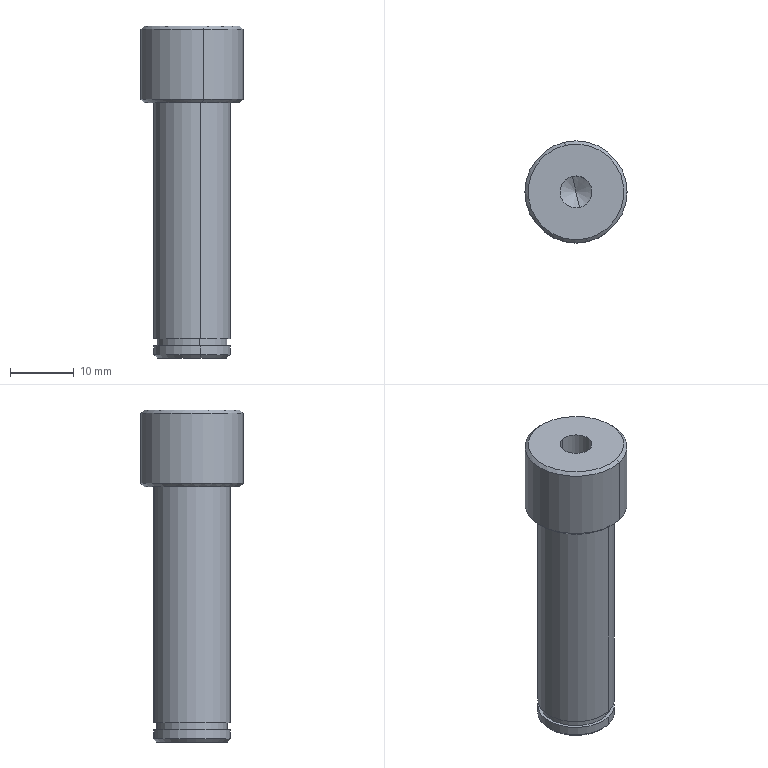Component | SolidWorks | JYTBJ-HeaderBrakeAxis-1 | 1 solid | 23 faces | box 16 x 16 x 52 mm | volume 6556 mm3 | cylinder 10 | cone 8 | plane 5 | commonest cylinder face diameters 12 x4 11 x2 5 x2 16 x2 | material AISI 1045 Steel, Cold Drawn
build123d program:
from build123d import *

# Parameters (mm, degrees)
SKETCH1_R             = 6
BOSS_EXTRUDE1_DEPTH   = 20
SKETCH2_R             = 8
BOSS_EXTRUDE2_DEPTH   = 12
M6_TAPPED_HOLE1_D     = 5
M6_TAPPED_HOLE1_DEPTH = 17
M6_TAPPED_HOLE1_TIP   = 1.502
SKETCH6_W             = 8.155
SKETCH6_H             = 1.1
CHAMFER1_SIZE         = 0.5


with BuildPart() as part:
    # Sketch1 → Boss-Extrude1 (new, symmetric)
    with BuildSketch(Plane.XY):
        Circle(SKETCH1_R)
    extrude(amount=BOSS_EXTRUDE1_DEPTH, both=True)

    # Sketch2 → Boss-Extrude2 (add)
    with BuildSketch(Plane.XY.offset(20)):
        Circle(SKETCH2_R)
    extrude(amount=BOSS_EXTRUDE2_DEPTH)

    # M6 Tapped Hole1
    with Locations(Plane(origin=(-7.558, 9.246, 32), x_dir=(1, 0, 0), z_dir=(0, 0, 1))):
        with Locations((7.558, -9.246)):
            Hole(M6_TAPPED_HOLE1_D / 2, depth=M6_TAPPED_HOLE1_DEPTH)
            with Locations((0, 0, -(M6_TAPPED_HOLE1_DEPTH + M6_TAPPED_HOLE1_TIP / 2))):  # 118° drill point
                Cone(0, M6_TAPPED_HOLE1_D / 2, M6_TAPPED_HOLE1_TIP, mode=Mode.SUBTRACT)

    # Sketch6 → Cut-Revolve1 (revolve, cut)
    with BuildSketch(Plane(origin=(0, 0, 0), x_dir=(1, 0, 0), z_dir=(0, 1, 0))):
        with Locations((9.578, 17.55)):
            Rectangle(SKETCH6_W, SKETCH6_H)
    revolve(axis=Axis((0, 0, 20), (0, 0, -1)), mode=Mode.SUBTRACT)

    # Chamfer1
    chamfer1_edges = [part.edges().sort_by_distance(p)[0] for p in [
        (-6, 0, -20),
        (-8, 0, 20),
        (-8, 0, 32),
    ]]
    chamfer(chamfer1_edges, length=CHAMFER1_SIZE)


solid = part.part

# Placed as in the assembly
solid = solid.moved(Location((-71.627, 226.781, -21), (0, 0, 0)))
STEP:
#1=COLOUR_RGB('',0.7922,0.8196,0.9333);
#2=FILL_AREA_STYLE_COLOUR('',#1);
#3=FILL_AREA_STYLE('',(#2));
#4=SURFACE_STYLE_FILL_AREA(#3);
#5=SURFACE_SIDE_STYLE('',(#4));
#6=SURFACE_STYLE_USAGE(.BOTH.,#5);
#7=PRESENTATION_STYLE_ASSIGNMENT((#6));
#8=CARTESIAN_POINT('',(-2.868,9.139,-1.614));
#9=VERTEX_POINT('',#8);
#10=CARTESIAN_POINT('',(-2.772,8.717,-1.614));
#11=VERTEX_POINT('',#10);
#12=CARTESIAN_POINT('',(-2.82,8.928,-1.614));
#13=DIRECTION('',(-0.,0.,-1.));
#14=DIRECTION('',(0.2228,-0.9749,0.));
#15=AXIS2_PLACEMENT_3D('',#12,#13,#14);
#16=CIRCLE('',#15,0.2165);
#17=EDGE_CURVE('',#9,#11,#16,.T.);
#18=ORIENTED_EDGE('',*,*,#17,.F.);
#19=CARTESIAN_POINT('',(-2.873,9.159,-1.594));
#20=VERTEX_POINT('',#19);
#21=CARTESIAN_POINT('',(-2.873,9.159,-1.594));
#22=DIRECTION('',(-0.1576,0.6893,0.7071));
#23=VECTOR('',#22,39.37);
#24=LINE('',#21,#23);
#25=EDGE_CURVE('',#9,#20,#24,.T.);
#26=ORIENTED_EDGE('',*,*,#25,.T.);
#27=CARTESIAN_POINT('',(-2.767,8.698,-1.594));
#28=VERTEX_POINT('',#27);
#29=CARTESIAN_POINT('',(-2.82,8.928,-1.594));
#30=DIRECTION('',(0.,-0.,1.));
#31=DIRECTION('',(0.2228,-0.9749,0.));
#32=AXIS2_PLACEMENT_3D('',#29,#30,#31);
#33=CIRCLE('',#32,0.2362);
#34=EDGE_CURVE('',#28,#20,#33,.T.);
#35=ORIENTED_EDGE('',*,*,#34,.F.);
#36=CARTESIAN_POINT('',(-2.767,8.698,-1.594));
#37=DIRECTION('',(0.1576,-0.6893,0.7071));
#38=VECTOR('',#37,39.37);
#39=LINE('',#36,#38);
#40=EDGE_CURVE('',#11,#28,#39,.T.);
#41=ORIENTED_EDGE('',*,*,#40,.F.);
#42=EDGE_LOOP('',(#18,#26,#35,#41));
#43=FACE_OUTER_BOUND('',#42,.T.);
#44=CARTESIAN_POINT('',(-2.82,8.928,-1.594));
#45=DIRECTION('',(0.,-0.,1.));
#46=DIRECTION('',(0.2228,-0.9749,0.));
#47=AXIS2_PLACEMENT_3D('',#44,#45,#46);
#48=CONICAL_SURFACE('',#47,0.2362,0.7854);
#49=ADVANCED_FACE('',(#43),#48,.T.);
#50=CARTESIAN_POINT('',(-2.886,9.216,-0.03937));
#51=VERTEX_POINT('',#50);
#52=CARTESIAN_POINT('',(-2.754,8.641,-0.03937));
#53=VERTEX_POINT('',#52);
#54=CARTESIAN_POINT('',(-2.82,8.928,-0.03937));
#55=DIRECTION('',(-0.,0.,-1.));
#56=DIRECTION('',(0.2228,-0.9749,0.));
#57=AXIS2_PLACEMENT_3D('',#54,#55,#56);
#58=CIRCLE('',#57,0.2953);
#59=EDGE_CURVE('',#51,#53,#58,.T.);
#60=ORIENTED_EDGE('',*,*,#59,.F.);
#61=CARTESIAN_POINT('',(-2.89,9.235,-0.01969));
#62=VERTEX_POINT('',#61);
#63=CARTESIAN_POINT('',(-2.89,9.235,-0.01969));
#64=DIRECTION('',(-0.1576,0.6893,0.7071));
#65=VECTOR('',#64,39.37);
#66=LINE('',#63,#65);
#67=EDGE_CURVE('',#51,#62,#66,.T.);
#68=ORIENTED_EDGE('',*,*,#67,.T.);
#69=CARTESIAN_POINT('',(-2.75,8.621,-0.01969));
#70=VERTEX_POINT('',#69);
#71=CARTESIAN_POINT('',(-2.82,8.928,-0.01969));
#72=DIRECTION('',(0.,-0.,1.));
#73=DIRECTION('',(0.2228,-0.9749,0.));
#74=AXIS2_PLACEMENT_3D('',#71,#72,#73);
#75=CIRCLE('',#74,0.315);
#76=EDGE_CURVE('',#70,#62,#75,.T.);
#77=ORIENTED_EDGE('',*,*,#76,.F.);
#78=CARTESIAN_POINT('',(-2.75,8.621,-0.01969));
#79=DIRECTION('',(0.1576,-0.6893,0.7071));
#80=VECTOR('',#79,39.37);
#81=LINE('',#78,#80);
#82=EDGE_CURVE('',#53,#70,#81,.T.);
#83=ORIENTED_EDGE('',*,*,#82,.F.);
#84=EDGE_LOOP('',(#60,#68,#77,#83));
#85=FACE_OUTER_BOUND('',#84,.T.);
#86=CARTESIAN_POINT('',(-2.82,8.928,-0.01969));
#87=DIRECTION('',(0.,-0.,1.));
#88=DIRECTION('',(0.2228,-0.9749,0.));
#89=AXIS2_PLACEMENT_3D('',#86,#87,#88);
#90=CONICAL_SURFACE('',#89,0.315,0.7854);
#91=ADVANCED_FACE('',(#85),#90,.T.);
#92=CARTESIAN_POINT('',(-2.754,8.641,0.4331));
#93=VERTEX_POINT('',#92);
#94=CARTESIAN_POINT('',(-2.886,9.216,0.4331));
#95=VERTEX_POINT('',#94);
#96=CARTESIAN_POINT('',(-2.82,8.928,0.4331));
#97=DIRECTION('',(0.,-0.,1.));
#98=DIRECTION('',(0.2228,-0.9749,0.));
#99=AXIS2_PLACEMENT_3D('',#96,#97,#98);
#100=CIRCLE('',#99,0.2953);
#101=EDGE_CURVE('',#93,#95,#100,.T.);
#102=ORIENTED_EDGE('',*,*,#101,.F.);
#103=CARTESIAN_POINT('',(-2.75,8.621,0.4134));
#104=VERTEX_POINT('',#103);
#105=CARTESIAN_POINT('',(-2.754,8.641,0.4331));
#106=DIRECTION('',(0.1576,-0.6893,-0.7071));
#107=VECTOR('',#106,39.37);
#108=LINE('',#105,#107);
#109=EDGE_CURVE('',#93,#104,#108,.T.);
#110=ORIENTED_EDGE('',*,*,#109,.T.);
#111=CARTESIAN_POINT('',(-2.89,9.235,0.4134));
#112=VERTEX_POINT('',#111);
#113=CARTESIAN_POINT('',(-2.82,8.928,0.4134));
#114=DIRECTION('',(-0.,0.,-1.));
#115=DIRECTION('',(0.2228,-0.9749,0.));
#116=AXIS2_PLACEMENT_3D('',#113,#114,#115);
#117=CIRCLE('',#116,0.315);
#118=EDGE_CURVE('',#112,#104,#117,.T.);
#119=ORIENTED_EDGE('',*,*,#118,.F.);
#120=CARTESIAN_POINT('',(-2.886,9.216,0.4331));
#121=DIRECTION('',(-0.1576,0.6893,-0.7071));
#122=VECTOR('',#121,39.37);
#123=LINE('',#120,#122);
#124=EDGE_CURVE('',#95,#112,#123,.T.);
#125=ORIENTED_EDGE('',*,*,#124,.F.);
#126=EDGE_LOOP('',(#102,#110,#119,#125));
#127=FACE_OUTER_BOUND('',#126,.T.);
#128=CARTESIAN_POINT('',(-2.82,8.928,0.4331));
#129=DIRECTION('',(-0.,0.,-1.));
#130=DIRECTION('',(-0.2228,0.9749,0.));
#131=AXIS2_PLACEMENT_3D('',#128,#129,#130);
#132=CONICAL_SURFACE('',#131,0.2953,0.7854);
#133=ADVANCED_FACE('',(#127),#132,.T.);
#134=CARTESIAN_POINT('',(-2.873,9.159,-1.539));
#135=VERTEX_POINT('',#134);
#136=CARTESIAN_POINT('',(-2.767,8.698,-1.539));
#137=VERTEX_POINT('',#136);
#138=CARTESIAN_POINT('',(-2.82,8.928,-1.539));
#139=DIRECTION('',(-0.,0.,-1.));
#140=DIRECTION('',(-0.2228,0.9749,0.));
#141=AXIS2_PLACEMENT_3D('',#138,#139,#140);
#142=CIRCLE('',#141,0.2362);
#143=EDGE_CURVE('',#135,#137,#142,.T.);
#144=ORIENTED_EDGE('',*,*,#143,.T.);
#145=CARTESIAN_POINT('',(-2.767,8.698,-0.03937));
#146=DIRECTION('',(-0.,0.,-1.));
#147=VECTOR('',#146,39.37);
#148=LINE('',#145,#147);
#149=EDGE_CURVE('',#137,#28,#148,.T.);
#150=ORIENTED_EDGE('',*,*,#149,.T.);
#151=ORIENTED_EDGE('',*,*,#34,.T.);
#152=CARTESIAN_POINT('',(-2.873,9.159,-0.03937));
#153=DIRECTION('',(-0.,0.,-1.));
#154=VECTOR('',#153,39.37);
#155=LINE('',#152,#154);
#156=EDGE_CURVE('',#135,#20,#155,.T.);
#157=ORIENTED_EDGE('',*,*,#156,.F.);
#158=EDGE_LOOP('',(#144,#150,#151,#157));
#159=FACE_OUTER_BOUND('',#158,.T.);
#160=CARTESIAN_POINT('',(-2.82,8.928,-0.03937));
#161=DIRECTION('',(-0.,0.,-1.));
#162=DIRECTION('',(-0.2228,0.9749,0.));
#163=AXIS2_PLACEMENT_3D('',#160,#161,#162);
#164=CYLINDRICAL_SURFACE('',#163,0.2362);
#165=ADVANCED_FACE('',(#159),#164,.T.);
#166=CARTESIAN_POINT('',(-2.772,8.717,-1.539));
#167=VERTEX_POINT('',#166);
#168=CARTESIAN_POINT('',(-2.868,9.139,-1.539));
#169=VERTEX_POINT('',#168);
#170=CARTESIAN_POINT('',(-2.82,8.928,-1.539));
#171=DIRECTION('',(0.,-0.,1.));
#172=DIRECTION('',(0.2228,-0.9749,0.));
#173=AXIS2_PLACEMENT_3D('',#170,#171,#172);
#174=CIRCLE('',#173,0.2165);
#175=EDGE_CURVE('',#167,#169,#174,.T.);
#176=ORIENTED_EDGE('',*,*,#175,.T.);
#177=CARTESIAN_POINT('',(-2.868,9.139,-1.496));
#178=VERTEX_POINT('',#177);
#179=CARTESIAN_POINT('',(-2.868,9.139,-0.03937));
#180=DIRECTION('',(0.,-0.,1.));
#181=VECTOR('',#180,39.37);
#182=LINE('',#179,#181);
#183=EDGE_CURVE('',#169,#178,#182,.T.);
#184=ORIENTED_EDGE('',*,*,#183,.T.);
#185=CARTESIAN_POINT('',(-2.772,8.717,-1.496));
#186=VERTEX_POINT('',#185);
#187=CARTESIAN_POINT('',(-2.82,8.928,-1.496));
#188=DIRECTION('',(0.,-0.,1.));
#189=DIRECTION('',(0.2228,-0.9749,0.));
#190=AXIS2_PLACEMENT_3D('',#187,#188,#189);
#191=CIRCLE('',#190,0.2165);
#192=EDGE_CURVE('',#186,#178,#191,.T.);
#193=ORIENTED_EDGE('',*,*,#192,.F.);
#194=CARTESIAN_POINT('',(-2.772,8.717,-0.03937));
#195=DIRECTION('',(0.,-0.,1.));
#196=VECTOR('',#195,39.37);
#197=LINE('',#194,#196);
#198=EDGE_CURVE('',#167,#186,#197,.T.);
#199=ORIENTED_EDGE('',*,*,#198,.F.);
#200=EDGE_LOOP('',(#176,#184,#193,#199));
#201=FACE_OUTER_BOUND('',#200,.T.);
#202=CARTESIAN_POINT('',(-2.82,8.928,-0.03937));
#203=DIRECTION('',(0.,-0.,1.));
#204=DIRECTION('',(0.2228,-0.9749,0.));
#205=AXIS2_PLACEMENT_3D('',#202,#203,#204);
#206=CYLINDRICAL_SURFACE('',#205,0.2165);
#207=ADVANCED_FACE('',(#201),#206,.T.);
#208=CARTESIAN_POINT('',(-2.842,9.024,-0.2362));
#209=VERTEX_POINT('',#208);
#210=CARTESIAN_POINT('',(-2.798,8.832,-0.2362));
#211=VERTEX_POINT('',#210);
#212=CARTESIAN_POINT('',(-2.82,8.928,-0.2362));
#213=DIRECTION('',(0.,-0.,1.));
#214=DIRECTION('',(0.2228,-0.9749,0.));
#215=AXIS2_PLACEMENT_3D('',#212,#213,#214);
#216=CIRCLE('',#215,0.09843);
#217=EDGE_CURVE('',#209,#211,#216,.T.);
#218=ORIENTED_EDGE('',*,*,#217,.F.);
#219=CARTESIAN_POINT('',(-2.842,9.024,0.4331));
#220=VERTEX_POINT('',#219);
#221=CARTESIAN_POINT('',(-2.842,9.024,0.4331));
#222=DIRECTION('',(0.,-0.,1.));
#223=VECTOR('',#222,39.37);
#224=LINE('',#221,#223);
#225=EDGE_CURVE('',#209,#220,#224,.T.);
#226=ORIENTED_EDGE('',*,*,#225,.T.);
#227=CARTESIAN_POINT('',(-2.798,8.832,0.4331));
#228=VERTEX_POINT('',#227);
#229=CARTESIAN_POINT('',(-2.82,8.928,0.4331));
#230=DIRECTION('',(0.,-0.,1.));
#231=DIRECTION('',(0.2228,-0.9749,0.));
#232=AXIS2_PLACEMENT_3D('',#229,#230,#231);
#233=CIRCLE('',#232,0.09843);
#234=EDGE_CURVE('',#220,#228,#233,.T.);
#235=ORIENTED_EDGE('',*,*,#234,.T.);
#236=CARTESIAN_POINT('',(-2.798,8.832,0.4331));
#237=DIRECTION('',(0.,-0.,1.));
#238=VECTOR('',#237,39.37);
#239=LINE('',#236,#238);
#240=EDGE_CURVE('',#211,#228,#239,.T.);
#241=ORIENTED_EDGE('',*,*,#240,.F.);
#242=EDGE_LOOP('',(#218,#226,#235,#241));
#243=FACE_OUTER_BOUND('',#242,.T.);
#244=CARTESIAN_POINT('',(-2.82,8.928,0.4331));
#245=DIRECTION('',(0.,-0.,1.));
#246=DIRECTION('',(0.2228,-0.9749,0.));
#247=AXIS2_PLACEMENT_3D('',#244,#245,#246);
#248=CYLINDRICAL_SURFACE('',#247,0.09843);
#249=ADVANCED_FACE('',(#243),#248,.F.);
#250=CARTESIAN_POINT('',(-2.82,8.928,-0.2954));
#251=VERTEX_POINT('',#250);
#252=CARTESIAN_POINT('',(-2.798,8.832,-0.2362));
#253=DIRECTION('',(0.191,-0.8356,0.515));
#254=VECTOR('',#253,39.37);
#255=LINE('',#252,#254);
#256=EDGE_CURVE('',#251,#211,#255,.T.);
#257=ORIENTED_EDGE('',*,*,#256,.F.);
#258=CARTESIAN_POINT('',(-2.842,9.024,-0.2362));
#259=DIRECTION('',(-0.191,0.8356,0.515));
#260=VECTOR('',#259,39.37);
#261=LINE('',#258,#260);
#262=EDGE_CURVE('',#251,#209,#261,.T.);
#263=ORIENTED_EDGE('',*,*,#262,.T.);
#264=ORIENTED_EDGE('',*,*,#217,.T.);
#265=EDGE_LOOP('',(#257,#263,#264));
#266=FACE_OUTER_BOUND('',#265,.T.);
#267=CARTESIAN_POINT('',(-2.82,8.928,-0.2362));
#268=DIRECTION('',(0.,-0.,1.));
#269=DIRECTION('',(0.2228,-0.9749,0.));
#270=AXIS2_PLACEMENT_3D('',#267,#268,#269);
#271=CONICAL_SURFACE('',#270,0.09843,1.03);
#272=ADVANCED_FACE('',(#266),#271,.F.);
#273=ORIENTED_EDGE('',*,*,#118,.T.);
#274=CARTESIAN_POINT('',(-2.75,8.621,0.4331));
#275=DIRECTION('',(-0.,0.,-1.));
#276=VECTOR('',#275,39.37);
#277=LINE('',#274,#276);
#278=EDGE_CURVE('',#104,#70,#277,.T.);
#279=ORIENTED_EDGE('',*,*,#278,.T.);
#280=ORIENTED_EDGE('',*,*,#76,.T.);
#281=CARTESIAN_POINT('',(-2.89,9.235,0.4331));
#282=DIRECTION('',(-0.,0.,-1.));
#283=VECTOR('',#282,39.37);
#284=LINE('',#281,#283);
#285=EDGE_CURVE('',#112,#62,#284,.T.);
#286=ORIENTED_EDGE('',*,*,#285,.F.);
#287=EDGE_LOOP('',(#273,#279,#280,#286));
#288=FACE_OUTER_BOUND('',#287,.T.);
#289=CARTESIAN_POINT('',(-2.82,8.928,0.4331));
#290=DIRECTION('',(-0.,0.,-1.));
#291=DIRECTION('',(-0.2228,0.9749,0.));
#292=AXIS2_PLACEMENT_3D('',#289,#290,#291);
#293=CYLINDRICAL_SURFACE('',#292,0.315);
#294=ADVANCED_FACE('',(#288),#293,.T.);
#295=CARTESIAN_POINT('',(-2.767,8.698,-0.03937));
#296=VERTEX_POINT('',#295);
#297=CARTESIAN_POINT('',(-2.873,9.159,-0.03937));
#298=VERTEX_POINT('',#297);
#299=CARTESIAN_POINT('',(-2.82,8.928,-0.03937));
#300=DIRECTION('',(0.,-0.,1.));
#301=DIRECTION('',(0.2228,-0.9749,0.));
#302=AXIS2_PLACEMENT_3D('',#299,#300,#301);
#303=CIRCLE('',#302,0.2362);
#304=EDGE_CURVE('',#296,#298,#303,.T.);
#305=ORIENTED_EDGE('',*,*,#304,.F.);
#306=CARTESIAN_POINT('',(-2.767,8.698,-1.496));
#307=VERTEX_POINT('',#306);
#308=CARTESIAN_POINT('',(-2.767,8.698,-0.03937));
#309=DIRECTION('',(-0.,0.,-1.));
#310=VECTOR('',#309,39.37);
#311=LINE('',#308,#310);
#312=EDGE_CURVE('',#296,#307,#311,.T.);
#313=ORIENTED_EDGE('',*,*,#312,.T.);
#314=CARTESIAN_POINT('',(-2.873,9.159,-1.496));
#315=VERTEX_POINT('',#314);
#316=CARTESIAN_POINT('',(-2.82,8.928,-1.496));
#317=DIRECTION('',(0.,-0.,1.));
#318=DIRECTION('',(0.2228,-0.9749,0.));
#319=AXIS2_PLACEMENT_3D('',#316,#317,#318);
#320=CIRCLE('',#319,0.2362);
#321=EDGE_CURVE('',#307,#315,#320,.T.);
#322=ORIENTED_EDGE('',*,*,#321,.T.);
#323=CARTESIAN_POINT('',(-2.873,9.159,-0.03937));
#324=DIRECTION('',(-0.,0.,-1.));
#325=VECTOR('',#324,39.37);
#326=LINE('',#323,#325);
#327=EDGE_CURVE('',#298,#315,#326,.T.);
#328=ORIENTED_EDGE('',*,*,#327,.F.);
#329=EDGE_LOOP('',(#305,#313,#322,#328));
#330=FACE_OUTER_BOUND('',#329,.T.);
#331=CARTESIAN_POINT('',(-2.82,8.928,-0.03937));
#332=DIRECTION('',(-0.,0.,-1.));
#333=DIRECTION('',(-0.2228,0.9749,0.));
#334=AXIS2_PLACEMENT_3D('',#331,#332,#333);
#335=CYLINDRICAL_SURFACE('',#334,0.2362);
#336=ADVANCED_FACE('',(#330),#335,.T.);
#337=ORIENTED_EDGE('',*,*,#312,.F.);
#338=CARTESIAN_POINT('',(-2.82,8.928,-0.03937));
#339=DIRECTION('',(0.,-0.,1.));
#340=DIRECTION('',(0.2228,-0.9749,0.));
#341=AXIS2_PLACEMENT_3D('',#338,#339,#340);
#342=CIRCLE('',#341,0.2362);
#343=EDGE_CURVE('',#298,#296,#342,.T.);
#344=ORIENTED_EDGE('',*,*,#343,.F.);
#345=ORIENTED_EDGE('',*,*,#327,.T.);
#346=CARTESIAN_POINT('',(-2.82,8.928,-1.496));
#347=DIRECTION('',(0.,-0.,1.));
#348=DIRECTION('',(0.2228,-0.9749,0.));
#349=AXIS2_PLACEMENT_3D('',#346,#347,#348);
#350=CIRCLE('',#349,0.2362);
#351=EDGE_CURVE('',#315,#307,#350,.T.);
#352=ORIENTED_EDGE('',*,*,#351,.T.);
#353=EDGE_LOOP('',(#337,#344,#345,#352));
#354=FACE_OUTER_BOUND('',#353,.T.);
#355=CARTESIAN_POINT('',(-2.82,8.928,-0.03937));
#356=DIRECTION('',(-0.,0.,-1.));
#357=DIRECTION('',(-0.2228,0.9749,0.));
#358=AXIS2_PLACEMENT_3D('',#355,#356,#357);
#359=CYLINDRICAL_SURFACE('',#358,0.2362);
#360=ADVANCED_FACE('',(#354),#359,.T.);
#361=CARTESIAN_POINT('',(-2.82,8.928,-0.03937));
#362=DIRECTION('',(-0.,0.,-1.));
#363=DIRECTION('',(0.2228,-0.9749,0.));
#364=AXIS2_PLACEMENT_3D('',#361,#362,#363);
#365=CIRCLE('',#364,0.2953);
#366=EDGE_CURVE('',#53,#51,#365,.T.);
#367=ORIENTED_EDGE('',*,*,#366,.T.);
#368=ORIENTED_EDGE('',*,*,#59,.T.);
#369=EDGE_LOOP('',(#367,#368));
#370=FACE_OUTER_BOUND('',#369,.T.);
#371=ORIENTED_EDGE('',*,*,#343,.T.);
#372=ORIENTED_EDGE('',*,*,#304,.T.);
#373=EDGE_LOOP('',(#371,#372));
#374=FACE_BOUND('',#373,.T.);
#375=CARTESIAN_POINT('',(-2.82,8.928,-0.03937));
#376=DIRECTION('',(0.,-0.,1.));
#377=DIRECTION('',(0.2228,-0.9749,-0.));
#378=AXIS2_PLACEMENT_3D('',#375,#376,#377);
#379=PLANE('',#378);
#380=ADVANCED_FACE('',(#370,#374),#379,.F.);
#381=ORIENTED_EDGE('',*,*,#278,.F.);
#382=CARTESIAN_POINT('',(-2.82,8.928,0.4134));
#383=DIRECTION('',(-0.,0.,-1.));
#384=DIRECTION('',(0.2228,-0.9749,0.));
#385=AXIS2_PLACEMENT_3D('',#382,#383,#384);
#386=CIRCLE('',#385,0.315);
#387=EDGE_CURVE('',#104,#112,#386,.T.);
#388=ORIENTED_EDGE('',*,*,#387,.T.);
#389=ORIENTED_EDGE('',*,*,#285,.T.);
#390=CARTESIAN_POINT('',(-2.82,8.928,-0.01969));
#391=DIRECTION('',(0.,-0.,1.));
#392=DIRECTION('',(0.2228,-0.9749,0.));
#393=AXIS2_PLACEMENT_3D('',#390,#391,#392);
#394=CIRCLE('',#393,0.315);
#395=EDGE_CURVE('',#62,#70,#394,.T.);
#396=ORIENTED_EDGE('',*,*,#395,.T.);
#397=EDGE_LOOP('',(#381,#388,#389,#396));
#398=FACE_OUTER_BOUND('',#397,.T.);
#399=CARTESIAN_POINT('',(-2.82,8.928,0.4331));
#400=DIRECTION('',(-0.,0.,-1.));
#401=DIRECTION('',(-0.2228,0.9749,0.));
#402=AXIS2_PLACEMENT_3D('',#399,#400,#401);
#403=CYLINDRICAL_SURFACE('',#402,0.315);
#404=ADVANCED_FACE('',(#398),#403,.T.);
#405=CARTESIAN_POINT('',(-2.82,8.928,0.4331));
#406=DIRECTION('',(0.,-0.,1.));
#407=DIRECTION('',(0.2228,-0.9749,0.));
#408=AXIS2_PLACEMENT_3D('',#405,#406,#407);
#409=CIRCLE('',#408,0.2953);
#410=EDGE_CURVE('',#95,#93,#409,.T.);
#411=ORIENTED_EDGE('',*,*,#410,.T.);
#412=ORIENTED_EDGE('',*,*,#101,.T.);
#413=EDGE_LOOP('',(#411,#412));
#414=FACE_OUTER_BOUND('',#413,.T.);
#415=CARTESIAN_POINT('',(-2.82,8.928,0.4331));
#416=DIRECTION('',(0.,-0.,1.));
#417=DIRECTION('',(0.2228,-0.9749,0.));
#418=AXIS2_PLACEMENT_3D('',#415,#416,#417);
#419=CIRCLE('',#418,0.09843);
#420=EDGE_CURVE('',#228,#220,#419,.T.);
#421=ORIENTED_EDGE('',*,*,#420,.F.);
#422=ORIENTED_EDGE('',*,*,#234,.F.);
#423=EDGE_LOOP('',(#421,#422));
#424=FACE_BOUND('',#423,.T.);
#425=CARTESIAN_POINT('',(-2.82,8.928,0.4331));
#426=DIRECTION('',(0.,-0.,1.));
#427=DIRECTION('',(0.2228,-0.9749,-0.));
#428=AXIS2_PLACEMENT_3D('',#425,#426,#427);
#429=PLANE('',#428);
#430=ADVANCED_FACE('',(#414,#424),#429,.T.);
#431=ORIENTED_EDGE('',*,*,#262,.F.);
#432=ORIENTED_EDGE('',*,*,#256,.T.);
#433=CARTESIAN_POINT('',(-2.82,8.928,-0.2362));
#434=DIRECTION('',(0.,-0.,1.));
#435=DIRECTION('',(0.2228,-0.9749,0.));
#436=AXIS2_PLACEMENT_3D('',#433,#434,#435);
#437=CIRCLE('',#436,0.09843);
#438=EDGE_CURVE('',#211,#209,#437,.T.);
#439=ORIENTED_EDGE('',*,*,#438,.T.);
#440=EDGE_LOOP('',(#431,#432,#439));
#441=FACE_OUTER_BOUND('',#440,.T.);
#442=CARTESIAN_POINT('',(-2.82,8.928,-0.2362));
#443=DIRECTION('',(0.,-0.,1.));
#444=DIRECTION('',(0.2228,-0.9749,0.));
#445=AXIS2_PLACEMENT_3D('',#442,#443,#444);
#446=CONICAL_SURFACE('',#445,0.09843,1.03);
#447=ADVANCED_FACE('',(#441),#446,.F.);
#448=ORIENTED_EDGE('',*,*,#225,.F.);
#449=ORIENTED_EDGE('',*,*,#438,.F.);
#450=ORIENTED_EDGE('',*,*,#240,.T.);
#451=ORIENTED_EDGE('',*,*,#420,.T.);
#452=EDGE_LOOP('',(#448,#449,#450,#451));
#453=FACE_OUTER_BOUND('',#452,.T.);
#454=CARTESIAN_POINT('',(-2.82,8.928,0.4331));
#455=DIRECTION('',(0.,-0.,1.));
#456=DIRECTION('',(0.2228,-0.9749,0.));
#457=AXIS2_PLACEMENT_3D('',#454,#455,#456);
#458=CYLINDRICAL_SURFACE('',#457,0.09843);
#459=ADVANCED_FACE('',(#453),#458,.F.);
#460=ORIENTED_EDGE('',*,*,#192,.T.);
#461=CARTESIAN_POINT('',(-2.82,8.928,-1.496));
#462=DIRECTION('',(0.,-0.,1.));
#463=DIRECTION('',(0.2228,-0.9749,0.));
#464=AXIS2_PLACEMENT_3D('',#461,#462,#463);
#465=CIRCLE('',#464,0.2165);
#466=EDGE_CURVE('',#178,#186,#465,.T.);
#467=ORIENTED_EDGE('',*,*,#466,.T.);
#468=EDGE_LOOP('',(#460,#467));
#469=FACE_BOUND('',#468,.T.);
#470=ORIENTED_EDGE('',*,*,#351,.F.);
#471=ORIENTED_EDGE('',*,*,#321,.F.);
#472=EDGE_LOOP('',(#470,#471));
#473=FACE_OUTER_BOUND('',#472,.T.);
#474=CARTESIAN_POINT('',(-2.772,8.717,-1.496));
#475=DIRECTION('',(0.,-0.,1.));
#476=DIRECTION('',(0.2228,-0.9749,-0.));
#477=AXIS2_PLACEMENT_3D('',#474,#475,#476);
#478=PLANE('',#477);
#479=ADVANCED_FACE('',(#469,#473),#478,.F.);
#480=ORIENTED_EDGE('',*,*,#175,.F.);
#481=CARTESIAN_POINT('',(-2.82,8.928,-1.539));
#482=DIRECTION('',(0.,-0.,1.));
#483=DIRECTION('',(0.2228,-0.9749,0.));
#484=AXIS2_PLACEMENT_3D('',#481,#482,#483);
#485=CIRCLE('',#484,0.2165);
#486=EDGE_CURVE('',#169,#167,#485,.T.);
#487=ORIENTED_EDGE('',*,*,#486,.F.);
#488=EDGE_LOOP('',(#480,#487));
#489=FACE_BOUND('',#488,.T.);
#490=ORIENTED_EDGE('',*,*,#143,.F.);
#491=CARTESIAN_POINT('',(-2.82,8.928,-1.539));
#492=DIRECTION('',(-0.,0.,-1.));
#493=DIRECTION('',(-0.2228,0.9749,0.));
#494=AXIS2_PLACEMENT_3D('',#491,#492,#493);
#495=CIRCLE('',#494,0.2362);
#496=EDGE_CURVE('',#137,#135,#495,.T.);
#497=ORIENTED_EDGE('',*,*,#496,.F.);
#498=EDGE_LOOP('',(#490,#497));
#499=FACE_OUTER_BOUND('',#498,.T.);
#500=CARTESIAN_POINT('',(-2.772,8.717,-1.539));
#501=DIRECTION('',(-0.,0.,-1.));
#502=DIRECTION('',(-0.2228,0.9749,0.));
#503=AXIS2_PLACEMENT_3D('',#500,#501,#502);
#504=PLANE('',#503);
#505=ADVANCED_FACE('',(#489,#499),#504,.F.);
#506=ORIENTED_EDGE('',*,*,#183,.F.);
#507=ORIENTED_EDGE('',*,*,#486,.T.);
#508=ORIENTED_EDGE('',*,*,#198,.T.);
#509=ORIENTED_EDGE('',*,*,#466,.F.);
#510=EDGE_LOOP('',(#506,#507,#508,#509));
#511=FACE_OUTER_BOUND('',#510,.T.);
#512=CARTESIAN_POINT('',(-2.82,8.928,-0.03937));
#513=DIRECTION('',(0.,-0.,1.));
#514=DIRECTION('',(0.2228,-0.9749,0.));
#515=AXIS2_PLACEMENT_3D('',#512,#513,#514);
#516=CYLINDRICAL_SURFACE('',#515,0.2165);
#517=ADVANCED_FACE('',(#511),#516,.T.);
#518=CARTESIAN_POINT('',(-2.82,8.928,-1.614));
#519=DIRECTION('',(-0.,0.,-1.));
#520=DIRECTION('',(0.2228,-0.9749,0.));
#521=AXIS2_PLACEMENT_3D('',#518,#519,#520);
#522=CIRCLE('',#521,0.2165);
#523=EDGE_CURVE('',#11,#9,#522,.T.);
#524=ORIENTED_EDGE('',*,*,#523,.T.);
#525=ORIENTED_EDGE('',*,*,#17,.T.);
#526=EDGE_LOOP('',(#524,#525));
#527=FACE_OUTER_BOUND('',#526,.T.);
#528=CARTESIAN_POINT('',(-2.82,8.928,-1.614));
#529=DIRECTION('',(0.,-0.,1.));
#530=DIRECTION('',(0.2228,-0.9749,-0.));
#531=AXIS2_PLACEMENT_3D('',#528,#529,#530);
#532=PLANE('',#531);
#533=ADVANCED_FACE('',(#527),#532,.F.);
#534=ORIENTED_EDGE('',*,*,#149,.F.);
#535=ORIENTED_EDGE('',*,*,#496,.T.);
#536=ORIENTED_EDGE('',*,*,#156,.T.);
#537=CARTESIAN_POINT('',(-2.82,8.928,-1.594));
#538=DIRECTION('',(0.,-0.,1.));
#539=DIRECTION('',(0.2228,-0.9749,0.));
#540=AXIS2_PLACEMENT_3D('',#537,#538,#539);
#541=CIRCLE('',#540,0.2362);
#542=EDGE_CURVE('',#20,#28,#541,.T.);
#543=ORIENTED_EDGE('',*,*,#542,.T.);
#544=EDGE_LOOP('',(#534,#535,#536,#543));
#545=FACE_OUTER_BOUND('',#544,.T.);
#546=CARTESIAN_POINT('',(-2.82,8.928,-0.03937));
#547=DIRECTION('',(-0.,0.,-1.));
#548=DIRECTION('',(-0.2228,0.9749,0.));
#549=AXIS2_PLACEMENT_3D('',#546,#547,#548);
#550=CYLINDRICAL_SURFACE('',#549,0.2362);
#551=ADVANCED_FACE('',(#545),#550,.T.);
#552=ORIENTED_EDGE('',*,*,#109,.F.);
#553=ORIENTED_EDGE('',*,*,#410,.F.);
#554=ORIENTED_EDGE('',*,*,#124,.T.);
#555=ORIENTED_EDGE('',*,*,#387,.F.);
#556=EDGE_LOOP('',(#552,#553,#554,#555));
#557=FACE_OUTER_BOUND('',#556,.T.);
#558=CARTESIAN_POINT('',(-2.82,8.928,0.4331));
#559=DIRECTION('',(-0.,0.,-1.));
#560=DIRECTION('',(-0.2228,0.9749,0.));
#561=AXIS2_PLACEMENT_3D('',#558,#559,#560);
#562=CONICAL_SURFACE('',#561,0.2953,0.7854);
#563=ADVANCED_FACE('',(#557),#562,.T.);
#564=ORIENTED_EDGE('',*,*,#67,.F.);
#565=ORIENTED_EDGE('',*,*,#366,.F.);
#566=ORIENTED_EDGE('',*,*,#82,.T.);
#567=ORIENTED_EDGE('',*,*,#395,.F.);
#568=EDGE_LOOP('',(#564,#565,#566,#567));
#569=FACE_OUTER_BOUND('',#568,.T.);
#570=CARTESIAN_POINT('',(-2.82,8.928,-0.01969));
#571=DIRECTION('',(0.,-0.,1.));
#572=DIRECTION('',(0.2228,-0.9749,0.));
#573=AXIS2_PLACEMENT_3D('',#570,#571,#572);
#574=CONICAL_SURFACE('',#573,0.315,0.7854);
#575=ADVANCED_FACE('',(#569),#574,.T.);
#576=ORIENTED_EDGE('',*,*,#25,.F.);
#577=ORIENTED_EDGE('',*,*,#523,.F.);
#578=ORIENTED_EDGE('',*,*,#40,.T.);
#579=ORIENTED_EDGE('',*,*,#542,.F.);
#580=EDGE_LOOP('',(#576,#577,#578,#579));
#581=FACE_OUTER_BOUND('',#580,.T.);
#582=CARTESIAN_POINT('',(-2.82,8.928,-1.594));
#583=DIRECTION('',(0.,-0.,1.));
#584=DIRECTION('',(0.2228,-0.9749,0.));
#585=AXIS2_PLACEMENT_3D('',#582,#583,#584);
#586=CONICAL_SURFACE('',#585,0.2362,0.7854);
#587=ADVANCED_FACE('',(#581),#586,.T.);
#588=CLOSED_SHELL('',(#49,#91,#133,#165,#207,#249,#272,#294,#336,#360,#380,#404,#430,#447,#459,#479,#505,#517,#533,#551,#563,#575,#587));
#589=MANIFOLD_SOLID_BREP('',#588);
#590=STYLED_ITEM('',(#7),#589);
#591=(LENGTH_UNIT()NAMED_UNIT(*)SI_UNIT($,.METRE.));
#592=LENGTH_MEASURE_WITH_UNIT(LENGTH_MEASURE(0.0254),#591);
#593=DIMENSIONAL_EXPONENTS(1.,0.,0.,0.,0.,0.,0.);
#594=(CONVERSION_BASED_UNIT('',#592)LENGTH_UNIT()NAMED_UNIT(#593));
#595=UNCERTAINTY_MEASURE_WITH_UNIT(LENGTH_MEASURE(0.00001),#594,'','');
#596=(NAMED_UNIT(*)PLANE_ANGLE_UNIT()SI_UNIT($,.RADIAN.));
#597=(NAMED_UNIT(*)SI_UNIT($,.STERADIAN.)SOLID_ANGLE_UNIT());
#598=(GEOMETRIC_REPRESENTATION_CONTEXT(3)GLOBAL_UNCERTAINTY_ASSIGNED_CONTEXT((#595))GLOBAL_UNIT_ASSIGNED_CONTEXT((#594,#596,#597))REPRESENTATION_CONTEXT('',''));
#599=MECHANICAL_DESIGN_GEOMETRIC_PRESENTATION_REPRESENTATION('',(#590),#598);
#600=PRESENTATION_LAYER_ASSIGNMENT('','',(#590));
#601=CARTESIAN_POINT('',(0.,0.,0.));
#602=DIRECTION('',(0.,0.,1.));
#603=DIRECTION('',(1.,0.,0.));
#604=AXIS2_PLACEMENT_3D('',#601,#602,#603);
#605=(LENGTH_UNIT()NAMED_UNIT(*)SI_UNIT($,.METRE.));
#606=LENGTH_MEASURE_WITH_UNIT(LENGTH_MEASURE(0.0254),#605);
#607=DIMENSIONAL_EXPONENTS(1.,0.,0.,0.,0.,0.,0.);
#608=(CONVERSION_BASED_UNIT('',#606)LENGTH_UNIT()NAMED_UNIT(#607));
#609=UNCERTAINTY_MEASURE_WITH_UNIT(LENGTH_MEASURE(0.00001),#608,'','');
#610=(NAMED_UNIT(*)PLANE_ANGLE_UNIT()SI_UNIT($,.RADIAN.));
#611=(NAMED_UNIT(*)SI_UNIT($,.STERADIAN.)SOLID_ANGLE_UNIT());
#612=(GEOMETRIC_REPRESENTATION_CONTEXT(3)GLOBAL_UNCERTAINTY_ASSIGNED_CONTEXT((#609))GLOBAL_UNIT_ASSIGNED_CONTEXT((#608,#610,#611))REPRESENTATION_CONTEXT('',''));
#613=ADVANCED_BREP_SHAPE_REPRESENTATION('',(#589,#604),#612);